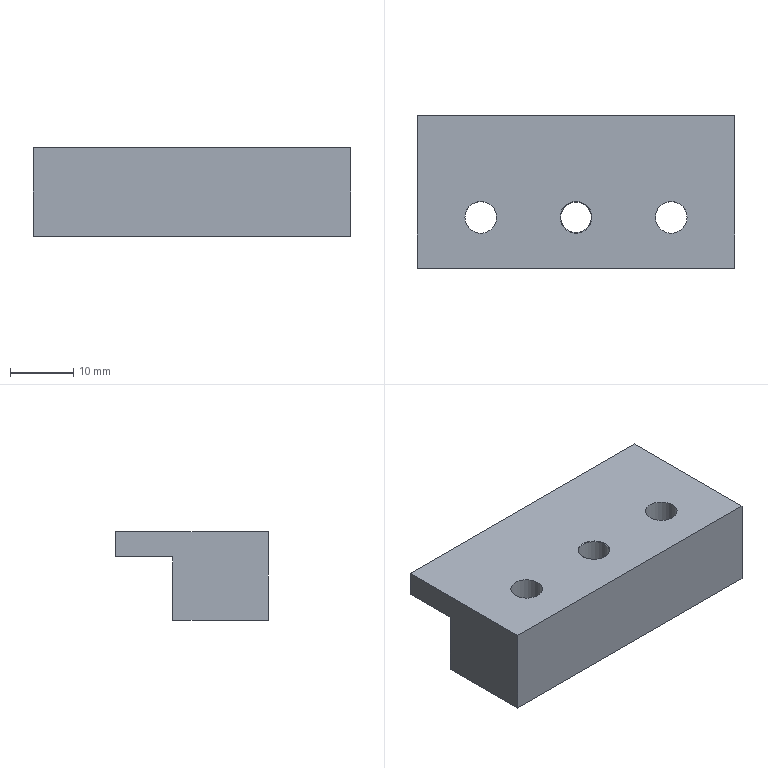Component | NX | GUIDE_PLATE_2 | 1 solid | 12 faces | box 50 x 24 x 14 mm | volume 11494 mm3 | plane 8 | cylinder 3 | cone 1 | commonest cylinder face diameters 5 x2 4.826 x1
STEP:
#1=CARTESIAN_POINT('',(0.,0.,0.));
#2=DIRECTION('',(0.,0.,1.));
#3=DIRECTION('',(1.,0.,0.));
#4=AXIS2_PLACEMENT_3D('',#1,#2,#3);
#5=CARTESIAN_POINT('',(28.,-11.,10.));
#6=VERTEX_POINT('',#5);
#7=CARTESIAN_POINT('',(28.,-11.,14.));
#8=VERTEX_POINT('',#7);
#9=CARTESIAN_POINT('',(28.,-11.,0.));
#10=DIRECTION('',(0.,0.,1.));
#11=VECTOR('',#10,1.);
#12=LINE('',#9,#11);
#13=CARTESIAN_POINT('',(28.,-11.,0.));
#14=DIRECTION('',(-0.,1.,0.));
#15=DIRECTION('',(-1.,-0.,0.));
#16=AXIS2_PLACEMENT_3D('',#13,#14,#15);
#17=PLANE('',#16);
#18=CARTESIAN_POINT('',(0.,0.));
#19=DIRECTION('',(0.,1.));
#20=VECTOR('',#19,1.);
#21=LINE('',#18,#20);
#22=(GEOMETRIC_REPRESENTATION_CONTEXT(2)PARAMETRIC_REPRESENTATION_CONTEXT()REPRESENTATION_CONTEXT('',''));
#23=DEFINITIONAL_REPRESENTATION('',(#21),#22);
#24=PCURVE('',#17,#23);
#25=CARTESIAN_POINT('',(28.,-35.,0.));
#26=DIRECTION('',(1.,0.,0.));
#27=DIRECTION('',(-0.,1.,0.));
#28=AXIS2_PLACEMENT_3D('',#25,#26,#27);
#29=PLANE('',#28);
#30=CARTESIAN_POINT('',(24.,0.));
#31=DIRECTION('',(0.,1.));
#32=VECTOR('',#31,1.);
#33=LINE('',#30,#32);
#34=(GEOMETRIC_REPRESENTATION_CONTEXT(2)PARAMETRIC_REPRESENTATION_CONTEXT()REPRESENTATION_CONTEXT('',''));
#35=DEFINITIONAL_REPRESENTATION('',(#33),#34);
#36=PCURVE('',#29,#35);
#37=SURFACE_CURVE('',#12,(#24,#36),.PCURVE_S1.);
#38=EDGE_CURVE('',#6,#8,#37,.T.);
#39=ORIENTED_EDGE('',*,*,#38,.F.);
#40=CARTESIAN_POINT('',(-22.,-11.,10.));
#41=VERTEX_POINT('',#40);
#42=CARTESIAN_POINT('',(55.,-11.,10.));
#43=DIRECTION('',(-1.,0.,0.));
#44=VECTOR('',#43,1.);
#45=LINE('',#42,#44);
#46=CARTESIAN_POINT('',(-27.,10.));
#47=DIRECTION('',(1.,0.));
#48=VECTOR('',#47,1.);
#49=LINE('',#46,#48);
#50=(GEOMETRIC_REPRESENTATION_CONTEXT(2)PARAMETRIC_REPRESENTATION_CONTEXT()REPRESENTATION_CONTEXT('',''));
#51=DEFINITIONAL_REPRESENTATION('',(#49),#50);
#52=PCURVE('',#17,#51);
#53=CARTESIAN_POINT('',(55.,-20.,10.));
#54=DIRECTION('',(0.,0.,1.));
#55=DIRECTION('',(0.,-1.,0.));
#56=AXIS2_PLACEMENT_3D('',#53,#54,#55);
#57=PLANE('',#56);
#58=CARTESIAN_POINT('',(-9.,0.));
#59=DIRECTION('',(0.,-1.));
#60=VECTOR('',#59,1.);
#61=LINE('',#58,#60);
#62=(GEOMETRIC_REPRESENTATION_CONTEXT(2)PARAMETRIC_REPRESENTATION_CONTEXT()REPRESENTATION_CONTEXT('',''));
#63=DEFINITIONAL_REPRESENTATION('',(#61),#62);
#64=PCURVE('',#57,#63);
#65=SURFACE_CURVE('',#45,(#52,#64),.PCURVE_S1.);
#66=EDGE_CURVE('',#6,#41,#65,.T.);
#67=ORIENTED_EDGE('',*,*,#66,.T.);
#68=CARTESIAN_POINT('',(-22.,-11.,14.));
#69=VERTEX_POINT('',#68);
#70=CARTESIAN_POINT('',(-22.,-11.,0.));
#71=DIRECTION('',(0.,0.,1.));
#72=VECTOR('',#71,1.);
#73=LINE('',#70,#72);
#74=CARTESIAN_POINT('',(50.,0.));
#75=DIRECTION('',(0.,1.));
#76=VECTOR('',#75,1.);
#77=LINE('',#74,#76);
#78=(GEOMETRIC_REPRESENTATION_CONTEXT(2)PARAMETRIC_REPRESENTATION_CONTEXT()REPRESENTATION_CONTEXT('',''));
#79=DEFINITIONAL_REPRESENTATION('',(#77),#78);
#80=PCURVE('',#17,#79);
#81=CARTESIAN_POINT('',(-22.,-11.,0.));
#82=DIRECTION('',(-1.,-0.,0.));
#83=DIRECTION('',(0.,-1.,0.));
#84=AXIS2_PLACEMENT_3D('',#81,#82,#83);
#85=PLANE('',#84);
#86=CARTESIAN_POINT('',(0.,0.));
#87=DIRECTION('',(0.,1.));
#88=VECTOR('',#87,1.);
#89=LINE('',#86,#88);
#90=(GEOMETRIC_REPRESENTATION_CONTEXT(2)PARAMETRIC_REPRESENTATION_CONTEXT()REPRESENTATION_CONTEXT('',''));
#91=DEFINITIONAL_REPRESENTATION('',(#89),#90);
#92=PCURVE('',#85,#91);
#93=SURFACE_CURVE('',#73,(#80,#92),.PCURVE_S1.);
#94=EDGE_CURVE('',#41,#69,#93,.T.);
#95=ORIENTED_EDGE('',*,*,#94,.T.);
#96=CARTESIAN_POINT('',(28.,-11.,14.));
#97=DIRECTION('',(-1.,-0.,0.));
#98=VECTOR('',#97,1.);
#99=LINE('',#96,#98);
#100=CARTESIAN_POINT('',(0.,14.));
#101=DIRECTION('',(1.,0.));
#102=VECTOR('',#101,1.);
#103=LINE('',#100,#102);
#104=(GEOMETRIC_REPRESENTATION_CONTEXT(2)PARAMETRIC_REPRESENTATION_CONTEXT()REPRESENTATION_CONTEXT('',''));
#105=DEFINITIONAL_REPRESENTATION('',(#103),#104);
#106=PCURVE('',#17,#105);
#107=CARTESIAN_POINT('',(-22.,-35.,14.));
#108=DIRECTION('',(0.,0.,1.));
#109=DIRECTION('',(1.,0.,0.));
#110=AXIS2_PLACEMENT_3D('',#107,#108,#109);
#111=PLANE('',#110);
#112=CARTESIAN_POINT('',(50.,24.));
#113=DIRECTION('',(-1.,-0.));
#114=VECTOR('',#113,1.);
#115=LINE('',#112,#114);
#116=(GEOMETRIC_REPRESENTATION_CONTEXT(2)PARAMETRIC_REPRESENTATION_CONTEXT()REPRESENTATION_CONTEXT('',''));
#117=DEFINITIONAL_REPRESENTATION('',(#115),#116);
#118=PCURVE('',#111,#117);
#119=SURFACE_CURVE('',#99,(#106,#118),.PCURVE_S1.);
#120=EDGE_CURVE('',#8,#69,#119,.T.);
#121=ORIENTED_EDGE('',*,*,#120,.F.);
#122=EDGE_LOOP('',(#39,#67,#95,#121));
#123=FACE_BOUND('',#122,.T.);
#124=ADVANCED_FACE('',(#123),#17,.T.);
#125=CARTESIAN_POINT('',(-9.5,-27.,0.));
#126=VERTEX_POINT('',#125);
#127=CARTESIAN_POINT('',(-14.5,-27.,0.));
#128=VERTEX_POINT('',#127);
#129=CARTESIAN_POINT('',(-12.,-27.,0.));
#130=DIRECTION('',(0.,0.,1.));
#131=DIRECTION('',(1.,0.,0.));
#132=AXIS2_PLACEMENT_3D('',#129,#130,#131);
#133=CIRCLE('',#132,2.5);
#134=CARTESIAN_POINT('',(-22.,-35.,0.));
#135=DIRECTION('',(0.,0.,1.));
#136=DIRECTION('',(1.,0.,0.));
#137=AXIS2_PLACEMENT_3D('',#134,#135,#136);
#138=PLANE('',#137);
#139=CARTESIAN_POINT('',(10.,8.));
#140=DIRECTION('',(1.,0.));
#141=AXIS2_PLACEMENT_2D('',#139,#140);
#142=CIRCLE('',#141,2.5);
#143=(GEOMETRIC_REPRESENTATION_CONTEXT(2)PARAMETRIC_REPRESENTATION_CONTEXT()REPRESENTATION_CONTEXT('',''));
#144=DEFINITIONAL_REPRESENTATION('',(#142),#143);
#145=PCURVE('',#138,#144);
#146=CARTESIAN_POINT('',(-12.,-27.,14.));
#147=DIRECTION('',(0.,0.,-1.));
#148=DIRECTION('',(-1.,0.,0.));
#149=AXIS2_PLACEMENT_3D('',#146,#147,#148);
#150=CYLINDRICAL_SURFACE('',#149,2.5);
#151=CARTESIAN_POINT('',(3.142,14.));
#152=DIRECTION('',(-1.,0.));
#153=VECTOR('',#152,1.);
#154=LINE('',#151,#153);
#155=(GEOMETRIC_REPRESENTATION_CONTEXT(2)PARAMETRIC_REPRESENTATION_CONTEXT()REPRESENTATION_CONTEXT('',''));
#156=DEFINITIONAL_REPRESENTATION('',(#154),#155);
#157=PCURVE('',#150,#156);
#158=SURFACE_CURVE('',#133,(#145,#157),.PCURVE_S1.);
#159=EDGE_CURVE('',#126,#128,#158,.T.);
#160=ORIENTED_EDGE('',*,*,#159,.T.);
#161=CARTESIAN_POINT('',(-12.,-27.,0.));
#162=DIRECTION('',(0.,0.,1.));
#163=DIRECTION('',(1.,0.,0.));
#164=AXIS2_PLACEMENT_3D('',#161,#162,#163);
#165=CIRCLE('',#164,2.5);
#166=CARTESIAN_POINT('',(10.,8.));
#167=DIRECTION('',(1.,0.));
#168=AXIS2_PLACEMENT_2D('',#166,#167);
#169=CIRCLE('',#168,2.5);
#170=(GEOMETRIC_REPRESENTATION_CONTEXT(2)PARAMETRIC_REPRESENTATION_CONTEXT()REPRESENTATION_CONTEXT('',''));
#171=DEFINITIONAL_REPRESENTATION('',(#169),#170);
#172=PCURVE('',#138,#171);
#173=CARTESIAN_POINT('',(9.425,14.));
#174=DIRECTION('',(-1.,0.));
#175=VECTOR('',#174,1.);
#176=LINE('',#173,#175);
#177=(GEOMETRIC_REPRESENTATION_CONTEXT(2)PARAMETRIC_REPRESENTATION_CONTEXT()REPRESENTATION_CONTEXT('',''));
#178=DEFINITIONAL_REPRESENTATION('',(#176),#177);
#179=PCURVE('',#150,#178);
#180=SURFACE_CURVE('',#165,(#172,#179),.PCURVE_S1.);
#181=EDGE_CURVE('',#128,#126,#180,.T.);
#182=ORIENTED_EDGE('',*,*,#181,.T.);
#183=EDGE_LOOP('',(#160,#182));
#184=FACE_BOUND('',#183,.T.);
#185=CARTESIAN_POINT('',(20.5,-27.,0.));
#186=VERTEX_POINT('',#185);
#187=CARTESIAN_POINT('',(15.5,-27.,0.));
#188=VERTEX_POINT('',#187);
#189=CARTESIAN_POINT('',(18.,-27.,0.));
#190=DIRECTION('',(0.,0.,1.));
#191=DIRECTION('',(1.,0.,0.));
#192=AXIS2_PLACEMENT_3D('',#189,#190,#191);
#193=CIRCLE('',#192,2.5);
#194=CARTESIAN_POINT('',(40.,8.));
#195=DIRECTION('',(1.,0.));
#196=AXIS2_PLACEMENT_2D('',#194,#195);
#197=CIRCLE('',#196,2.5);
#198=(GEOMETRIC_REPRESENTATION_CONTEXT(2)PARAMETRIC_REPRESENTATION_CONTEXT()REPRESENTATION_CONTEXT('',''));
#199=DEFINITIONAL_REPRESENTATION('',(#197),#198);
#200=PCURVE('',#138,#199);
#201=CARTESIAN_POINT('',(18.,-27.,14.));
#202=DIRECTION('',(0.,0.,-1.));
#203=DIRECTION('',(-1.,0.,0.));
#204=AXIS2_PLACEMENT_3D('',#201,#202,#203);
#205=CYLINDRICAL_SURFACE('',#204,2.5);
#206=CARTESIAN_POINT('',(3.142,14.));
#207=DIRECTION('',(-1.,0.));
#208=VECTOR('',#207,1.);
#209=LINE('',#206,#208);
#210=(GEOMETRIC_REPRESENTATION_CONTEXT(2)PARAMETRIC_REPRESENTATION_CONTEXT()REPRESENTATION_CONTEXT('',''));
#211=DEFINITIONAL_REPRESENTATION('',(#209),#210);
#212=PCURVE('',#205,#211);
#213=SURFACE_CURVE('',#193,(#200,#212),.PCURVE_S1.);
#214=EDGE_CURVE('',#186,#188,#213,.T.);
#215=ORIENTED_EDGE('',*,*,#214,.T.);
#216=CARTESIAN_POINT('',(18.,-27.,0.));
#217=DIRECTION('',(0.,0.,1.));
#218=DIRECTION('',(1.,0.,0.));
#219=AXIS2_PLACEMENT_3D('',#216,#217,#218);
#220=CIRCLE('',#219,2.5);
#221=CARTESIAN_POINT('',(40.,8.));
#222=DIRECTION('',(1.,0.));
#223=AXIS2_PLACEMENT_2D('',#221,#222);
#224=CIRCLE('',#223,2.5);
#225=(GEOMETRIC_REPRESENTATION_CONTEXT(2)PARAMETRIC_REPRESENTATION_CONTEXT()REPRESENTATION_CONTEXT('',''));
#226=DEFINITIONAL_REPRESENTATION('',(#224),#225);
#227=PCURVE('',#138,#226);
#228=CARTESIAN_POINT('',(9.425,14.));
#229=DIRECTION('',(-1.,0.));
#230=VECTOR('',#229,1.);
#231=LINE('',#228,#230);
#232=(GEOMETRIC_REPRESENTATION_CONTEXT(2)PARAMETRIC_REPRESENTATION_CONTEXT()REPRESENTATION_CONTEXT('',''));
#233=DEFINITIONAL_REPRESENTATION('',(#231),#232);
#234=PCURVE('',#205,#233);
#235=SURFACE_CURVE('',#220,(#227,#234),.PCURVE_S1.);
#236=EDGE_CURVE('',#188,#186,#235,.T.);
#237=ORIENTED_EDGE('',*,*,#236,.T.);
#238=EDGE_LOOP('',(#215,#237));
#239=FACE_BOUND('',#238,.T.);
#240=CARTESIAN_POINT('',(5.413,-27.,0.));
#241=VERTEX_POINT('',#240);
#242=CARTESIAN_POINT('',(3.,-27.,0.));
#243=DIRECTION('',(0.,0.,1.));
#244=DIRECTION('',(1.,0.,0.));
#245=AXIS2_PLACEMENT_3D('',#242,#243,#244);
#246=CIRCLE('',#245,2.413);
#247=CARTESIAN_POINT('',(25.,8.));
#248=DIRECTION('',(1.,0.));
#249=AXIS2_PLACEMENT_2D('',#247,#248);
#250=CIRCLE('',#249,2.413);
#251=(GEOMETRIC_REPRESENTATION_CONTEXT(2)PARAMETRIC_REPRESENTATION_CONTEXT()REPRESENTATION_CONTEXT('',''));
#252=DEFINITIONAL_REPRESENTATION('',(#250),#251);
#253=PCURVE('',#138,#252);
#254=CARTESIAN_POINT('',(3.,-27.,14.));
#255=DIRECTION('',(0.,0.,-1.));
#256=DIRECTION('',(-1.,0.,0.));
#257=AXIS2_PLACEMENT_3D('',#254,#255,#256);
#258=CYLINDRICAL_SURFACE('',#257,2.413);
#259=CARTESIAN_POINT('',(9.425,14.));
#260=DIRECTION('',(-1.,0.));
#261=VECTOR('',#260,1.);
#262=LINE('',#259,#261);
#263=(GEOMETRIC_REPRESENTATION_CONTEXT(2)PARAMETRIC_REPRESENTATION_CONTEXT()REPRESENTATION_CONTEXT('',''));
#264=DEFINITIONAL_REPRESENTATION('',(#262),#263);
#265=PCURVE('',#258,#264);
#266=SURFACE_CURVE('',#246,(#253,#265),.PCURVE_S1.);
#267=EDGE_CURVE('',#241,#241,#266,.T.);
#268=ORIENTED_EDGE('',*,*,#267,.T.);
#269=EDGE_LOOP('',(#268));
#270=FACE_BOUND('',#269,.T.);
#271=CARTESIAN_POINT('',(28.,-20.,0.));
#272=VERTEX_POINT('',#271);
#273=CARTESIAN_POINT('',(-22.,-20.,0.));
#274=VERTEX_POINT('',#273);
#275=CARTESIAN_POINT('',(55.,-20.,0.));
#276=DIRECTION('',(-1.,0.,0.));
#277=VECTOR('',#276,1.);
#278=LINE('',#275,#277);
#279=CARTESIAN_POINT('',(77.,15.));
#280=DIRECTION('',(-1.,0.));
#281=VECTOR('',#280,1.);
#282=LINE('',#279,#281);
#283=(GEOMETRIC_REPRESENTATION_CONTEXT(2)PARAMETRIC_REPRESENTATION_CONTEXT()REPRESENTATION_CONTEXT('',''));
#284=DEFINITIONAL_REPRESENTATION('',(#282),#283);
#285=PCURVE('',#138,#284);
#286=CARTESIAN_POINT('',(55.,-20.,0.));
#287=DIRECTION('',(0.,-1.,0.));
#288=DIRECTION('',(0.,-0.,-1.));
#289=AXIS2_PLACEMENT_3D('',#286,#287,#288);
#290=PLANE('',#289);
#291=CARTESIAN_POINT('',(0.,0.));
#292=DIRECTION('',(0.,-1.));
#293=VECTOR('',#292,1.);
#294=LINE('',#291,#293);
#295=(GEOMETRIC_REPRESENTATION_CONTEXT(2)PARAMETRIC_REPRESENTATION_CONTEXT()REPRESENTATION_CONTEXT('',''));
#296=DEFINITIONAL_REPRESENTATION('',(#294),#295);
#297=PCURVE('',#290,#296);
#298=SURFACE_CURVE('',#278,(#285,#297),.PCURVE_S1.);
#299=EDGE_CURVE('',#272,#274,#298,.T.);
#300=ORIENTED_EDGE('',*,*,#299,.F.);
#301=CARTESIAN_POINT('',(28.,-35.,0.));
#302=VERTEX_POINT('',#301);
#303=CARTESIAN_POINT('',(28.,-35.,0.));
#304=DIRECTION('',(-0.,1.,0.));
#305=VECTOR('',#304,1.);
#306=LINE('',#303,#305);
#307=CARTESIAN_POINT('',(50.,0.));
#308=DIRECTION('',(-0.,1.));
#309=VECTOR('',#308,1.);
#310=LINE('',#307,#309);
#311=(GEOMETRIC_REPRESENTATION_CONTEXT(2)PARAMETRIC_REPRESENTATION_CONTEXT()REPRESENTATION_CONTEXT('',''));
#312=DEFINITIONAL_REPRESENTATION('',(#310),#311);
#313=PCURVE('',#138,#312);
#314=CARTESIAN_POINT('',(0.,0.));
#315=DIRECTION('',(1.,0.));
#316=VECTOR('',#315,1.);
#317=LINE('',#314,#316);
#318=(GEOMETRIC_REPRESENTATION_CONTEXT(2)PARAMETRIC_REPRESENTATION_CONTEXT()REPRESENTATION_CONTEXT('',''));
#319=DEFINITIONAL_REPRESENTATION('',(#317),#318);
#320=PCURVE('',#29,#319);
#321=SURFACE_CURVE('',#306,(#313,#320),.PCURVE_S1.);
#322=EDGE_CURVE('',#302,#272,#321,.T.);
#323=ORIENTED_EDGE('',*,*,#322,.F.);
#324=CARTESIAN_POINT('',(-22.,-35.,0.));
#325=VERTEX_POINT('',#324);
#326=CARTESIAN_POINT('',(-22.,-35.,0.));
#327=DIRECTION('',(1.,-0.,0.));
#328=VECTOR('',#327,1.);
#329=LINE('',#326,#328);
#330=CARTESIAN_POINT('',(0.,0.));
#331=DIRECTION('',(1.,-0.));
#332=VECTOR('',#331,1.);
#333=LINE('',#330,#332);
#334=(GEOMETRIC_REPRESENTATION_CONTEXT(2)PARAMETRIC_REPRESENTATION_CONTEXT()REPRESENTATION_CONTEXT('',''));
#335=DEFINITIONAL_REPRESENTATION('',(#333),#334);
#336=PCURVE('',#138,#335);
#337=CARTESIAN_POINT('',(-22.,-35.,0.));
#338=DIRECTION('',(-0.,-1.,0.));
#339=DIRECTION('',(1.,-0.,0.));
#340=AXIS2_PLACEMENT_3D('',#337,#338,#339);
#341=PLANE('',#340);
#342=CARTESIAN_POINT('',(0.,0.));
#343=DIRECTION('',(1.,0.));
#344=VECTOR('',#343,1.);
#345=LINE('',#342,#344);
#346=(GEOMETRIC_REPRESENTATION_CONTEXT(2)PARAMETRIC_REPRESENTATION_CONTEXT()REPRESENTATION_CONTEXT('',''));
#347=DEFINITIONAL_REPRESENTATION('',(#345),#346);
#348=PCURVE('',#341,#347);
#349=SURFACE_CURVE('',#329,(#336,#348),.PCURVE_S1.);
#350=EDGE_CURVE('',#325,#302,#349,.T.);
#351=ORIENTED_EDGE('',*,*,#350,.F.);
#352=CARTESIAN_POINT('',(-22.,-11.,0.));
#353=DIRECTION('',(0.,-1.,0.));
#354=VECTOR('',#353,1.);
#355=LINE('',#352,#354);
#356=CARTESIAN_POINT('',(0.,24.));
#357=DIRECTION('',(0.,-1.));
#358=VECTOR('',#357,1.);
#359=LINE('',#356,#358);
#360=(GEOMETRIC_REPRESENTATION_CONTEXT(2)PARAMETRIC_REPRESENTATION_CONTEXT()REPRESENTATION_CONTEXT('',''));
#361=DEFINITIONAL_REPRESENTATION('',(#359),#360);
#362=PCURVE('',#138,#361);
#363=CARTESIAN_POINT('',(0.,0.));
#364=DIRECTION('',(1.,0.));
#365=VECTOR('',#364,1.);
#366=LINE('',#363,#365);
#367=(GEOMETRIC_REPRESENTATION_CONTEXT(2)PARAMETRIC_REPRESENTATION_CONTEXT()REPRESENTATION_CONTEXT('',''));
#368=DEFINITIONAL_REPRESENTATION('',(#366),#367);
#369=PCURVE('',#85,#368);
#370=SURFACE_CURVE('',#355,(#362,#369),.PCURVE_S1.);
#371=EDGE_CURVE('',#274,#325,#370,.T.);
#372=ORIENTED_EDGE('',*,*,#371,.F.);
#373=EDGE_LOOP('',(#300,#323,#351,#372));
#374=FACE_BOUND('',#373,.T.);
#375=ADVANCED_FACE('',(#184,#239,#270,#374),#138,.F.);
#376=CARTESIAN_POINT('',(-22.,-20.,10.));
#377=VERTEX_POINT('',#376);
#378=CARTESIAN_POINT('',(-22.,-20.,0.));
#379=DIRECTION('',(-0.,0.,1.));
#380=VECTOR('',#379,1.);
#381=LINE('',#378,#380);
#382=CARTESIAN_POINT('',(9.,0.));
#383=DIRECTION('',(-0.,1.));
#384=VECTOR('',#383,1.);
#385=LINE('',#382,#384);
#386=(GEOMETRIC_REPRESENTATION_CONTEXT(2)PARAMETRIC_REPRESENTATION_CONTEXT()REPRESENTATION_CONTEXT('',''));
#387=DEFINITIONAL_REPRESENTATION('',(#385),#386);
#388=PCURVE('',#85,#387);
#389=CARTESIAN_POINT('',(-0.,-77.));
#390=DIRECTION('',(-1.,-0.));
#391=VECTOR('',#390,1.);
#392=LINE('',#389,#391);
#393=(GEOMETRIC_REPRESENTATION_CONTEXT(2)PARAMETRIC_REPRESENTATION_CONTEXT()REPRESENTATION_CONTEXT('',''));
#394=DEFINITIONAL_REPRESENTATION('',(#392),#393);
#395=PCURVE('',#290,#394);
#396=SURFACE_CURVE('',#381,(#388,#395),.PCURVE_S1.);
#397=EDGE_CURVE('',#274,#377,#396,.T.);
#398=ORIENTED_EDGE('',*,*,#397,.F.);
#399=ORIENTED_EDGE('',*,*,#371,.T.);
#400=CARTESIAN_POINT('',(-22.,-35.,14.));
#401=VERTEX_POINT('',#400);
#402=CARTESIAN_POINT('',(-22.,-35.,0.));
#403=DIRECTION('',(0.,0.,1.));
#404=VECTOR('',#403,1.);
#405=LINE('',#402,#404);
#406=CARTESIAN_POINT('',(24.,0.));
#407=DIRECTION('',(0.,1.));
#408=VECTOR('',#407,1.);
#409=LINE('',#406,#408);
#410=(GEOMETRIC_REPRESENTATION_CONTEXT(2)PARAMETRIC_REPRESENTATION_CONTEXT()REPRESENTATION_CONTEXT('',''));
#411=DEFINITIONAL_REPRESENTATION('',(#409),#410);
#412=PCURVE('',#85,#411);
#413=CARTESIAN_POINT('',(0.,0.));
#414=DIRECTION('',(0.,1.));
#415=VECTOR('',#414,1.);
#416=LINE('',#413,#415);
#417=(GEOMETRIC_REPRESENTATION_CONTEXT(2)PARAMETRIC_REPRESENTATION_CONTEXT()REPRESENTATION_CONTEXT('',''));
#418=DEFINITIONAL_REPRESENTATION('',(#416),#417);
#419=PCURVE('',#341,#418);
#420=SURFACE_CURVE('',#405,(#412,#419),.PCURVE_S1.);
#421=EDGE_CURVE('',#325,#401,#420,.T.);
#422=ORIENTED_EDGE('',*,*,#421,.T.);
#423=CARTESIAN_POINT('',(-22.,-11.,14.));
#424=DIRECTION('',(0.,-1.,0.));
#425=VECTOR('',#424,1.);
#426=LINE('',#423,#425);
#427=CARTESIAN_POINT('',(0.,14.));
#428=DIRECTION('',(1.,0.));
#429=VECTOR('',#428,1.);
#430=LINE('',#427,#429);
#431=(GEOMETRIC_REPRESENTATION_CONTEXT(2)PARAMETRIC_REPRESENTATION_CONTEXT()REPRESENTATION_CONTEXT('',''));
#432=DEFINITIONAL_REPRESENTATION('',(#430),#431);
#433=PCURVE('',#85,#432);
#434=CARTESIAN_POINT('',(0.,24.));
#435=DIRECTION('',(0.,-1.));
#436=VECTOR('',#435,1.);
#437=LINE('',#434,#436);
#438=(GEOMETRIC_REPRESENTATION_CONTEXT(2)PARAMETRIC_REPRESENTATION_CONTEXT()REPRESENTATION_CONTEXT('',''));
#439=DEFINITIONAL_REPRESENTATION('',(#437),#438);
#440=PCURVE('',#111,#439);
#441=SURFACE_CURVE('',#426,(#433,#440),.PCURVE_S1.);
#442=EDGE_CURVE('',#69,#401,#441,.T.);
#443=ORIENTED_EDGE('',*,*,#442,.F.);
#444=ORIENTED_EDGE('',*,*,#94,.F.);
#445=CARTESIAN_POINT('',(-22.,-11.,10.));
#446=DIRECTION('',(-0.,1.,-0.));
#447=VECTOR('',#446,1.);
#448=LINE('',#445,#447);
#449=CARTESIAN_POINT('',(0.,10.));
#450=DIRECTION('',(-1.,-0.));
#451=VECTOR('',#450,1.);
#452=LINE('',#449,#451);
#453=(GEOMETRIC_REPRESENTATION_CONTEXT(2)PARAMETRIC_REPRESENTATION_CONTEXT()REPRESENTATION_CONTEXT('',''));
#454=DEFINITIONAL_REPRESENTATION('',(#452),#453);
#455=PCURVE('',#85,#454);
#456=CARTESIAN_POINT('',(-9.,-77.));
#457=DIRECTION('',(-1.,-0.));
#458=VECTOR('',#457,1.);
#459=LINE('',#456,#458);
#460=(GEOMETRIC_REPRESENTATION_CONTEXT(2)PARAMETRIC_REPRESENTATION_CONTEXT()REPRESENTATION_CONTEXT('',''));
#461=DEFINITIONAL_REPRESENTATION('',(#459),#460);
#462=PCURVE('',#57,#461);
#463=SURFACE_CURVE('',#448,(#455,#462),.PCURVE_S1.);
#464=EDGE_CURVE('',#377,#41,#463,.T.);
#465=ORIENTED_EDGE('',*,*,#464,.F.);
#466=EDGE_LOOP('',(#398,#399,#422,#443,#444,#465));
#467=FACE_BOUND('',#466,.T.);
#468=ADVANCED_FACE('',(#467),#85,.T.);
#469=CARTESIAN_POINT('',(28.,-35.,14.));
#470=VERTEX_POINT('',#469);
#471=CARTESIAN_POINT('',(-22.,-35.,14.));
#472=DIRECTION('',(1.,-0.,0.));
#473=VECTOR('',#472,1.);
#474=LINE('',#471,#473);
#475=CARTESIAN_POINT('',(0.,14.));
#476=DIRECTION('',(1.,0.));
#477=VECTOR('',#476,1.);
#478=LINE('',#475,#477);
#479=(GEOMETRIC_REPRESENTATION_CONTEXT(2)PARAMETRIC_REPRESENTATION_CONTEXT()REPRESENTATION_CONTEXT('',''));
#480=DEFINITIONAL_REPRESENTATION('',(#478),#479);
#481=PCURVE('',#341,#480);
#482=CARTESIAN_POINT('',(0.,0.));
#483=DIRECTION('',(1.,-0.));
#484=VECTOR('',#483,1.);
#485=LINE('',#482,#484);
#486=(GEOMETRIC_REPRESENTATION_CONTEXT(2)PARAMETRIC_REPRESENTATION_CONTEXT()REPRESENTATION_CONTEXT('',''));
#487=DEFINITIONAL_REPRESENTATION('',(#485),#486);
#488=PCURVE('',#111,#487);
#489=SURFACE_CURVE('',#474,(#481,#488),.PCURVE_S1.);
#490=EDGE_CURVE('',#401,#470,#489,.T.);
#491=ORIENTED_EDGE('',*,*,#490,.F.);
#492=ORIENTED_EDGE('',*,*,#421,.F.);
#493=ORIENTED_EDGE('',*,*,#350,.T.);
#494=CARTESIAN_POINT('',(28.,-35.,0.));
#495=DIRECTION('',(0.,0.,1.));
#496=VECTOR('',#495,1.);
#497=LINE('',#494,#496);
#498=CARTESIAN_POINT('',(50.,0.));
#499=DIRECTION('',(0.,1.));
#500=VECTOR('',#499,1.);
#501=LINE('',#498,#500);
#502=(GEOMETRIC_REPRESENTATION_CONTEXT(2)PARAMETRIC_REPRESENTATION_CONTEXT()REPRESENTATION_CONTEXT('',''));
#503=DEFINITIONAL_REPRESENTATION('',(#501),#502);
#504=PCURVE('',#341,#503);
#505=CARTESIAN_POINT('',(0.,0.));
#506=DIRECTION('',(0.,1.));
#507=VECTOR('',#506,1.);
#508=LINE('',#505,#507);
#509=(GEOMETRIC_REPRESENTATION_CONTEXT(2)PARAMETRIC_REPRESENTATION_CONTEXT()REPRESENTATION_CONTEXT('',''));
#510=DEFINITIONAL_REPRESENTATION('',(#508),#509);
#511=PCURVE('',#29,#510);
#512=SURFACE_CURVE('',#497,(#504,#511),.PCURVE_S1.);
#513=EDGE_CURVE('',#302,#470,#512,.T.);
#514=ORIENTED_EDGE('',*,*,#513,.T.);
#515=EDGE_LOOP('',(#491,#492,#493,#514));
#516=FACE_BOUND('',#515,.T.);
#517=ADVANCED_FACE('',(#516),#341,.T.);
#518=CARTESIAN_POINT('',(28.,-20.,10.));
#519=VERTEX_POINT('',#518);
#520=CARTESIAN_POINT('',(28.,-20.,-0.));
#521=DIRECTION('',(0.,-0.,-1.));
#522=VECTOR('',#521,1.);
#523=LINE('',#520,#522);
#524=CARTESIAN_POINT('',(15.,-0.));
#525=DIRECTION('',(-0.,-1.));
#526=VECTOR('',#525,1.);
#527=LINE('',#524,#526);
#528=(GEOMETRIC_REPRESENTATION_CONTEXT(2)PARAMETRIC_REPRESENTATION_CONTEXT()REPRESENTATION_CONTEXT('',''));
#529=DEFINITIONAL_REPRESENTATION('',(#527),#528);
#530=PCURVE('',#29,#529);
#531=CARTESIAN_POINT('',(0.,-27.));
#532=DIRECTION('',(1.,0.));
#533=VECTOR('',#532,1.);
#534=LINE('',#531,#533);
#535=(GEOMETRIC_REPRESENTATION_CONTEXT(2)PARAMETRIC_REPRESENTATION_CONTEXT()REPRESENTATION_CONTEXT('',''));
#536=DEFINITIONAL_REPRESENTATION('',(#534),#535);
#537=PCURVE('',#290,#536);
#538=SURFACE_CURVE('',#523,(#530,#537),.PCURVE_S1.);
#539=EDGE_CURVE('',#519,#272,#538,.T.);
#540=ORIENTED_EDGE('',*,*,#539,.F.);
#541=CARTESIAN_POINT('',(28.,-35.,10.));
#542=DIRECTION('',(0.,-1.,0.));
#543=VECTOR('',#542,1.);
#544=LINE('',#541,#543);
#545=CARTESIAN_POINT('',(0.,10.));
#546=DIRECTION('',(-1.,0.));
#547=VECTOR('',#546,1.);
#548=LINE('',#545,#547);
#549=(GEOMETRIC_REPRESENTATION_CONTEXT(2)PARAMETRIC_REPRESENTATION_CONTEXT()REPRESENTATION_CONTEXT('',''));
#550=DEFINITIONAL_REPRESENTATION('',(#548),#549);
#551=PCURVE('',#29,#550);
#552=CARTESIAN_POINT('',(15.,-27.));
#553=DIRECTION('',(1.,0.));
#554=VECTOR('',#553,1.);
#555=LINE('',#552,#554);
#556=(GEOMETRIC_REPRESENTATION_CONTEXT(2)PARAMETRIC_REPRESENTATION_CONTEXT()REPRESENTATION_CONTEXT('',''));
#557=DEFINITIONAL_REPRESENTATION('',(#555),#556);
#558=PCURVE('',#57,#557);
#559=SURFACE_CURVE('',#544,(#551,#558),.PCURVE_S1.);
#560=EDGE_CURVE('',#6,#519,#559,.T.);
#561=ORIENTED_EDGE('',*,*,#560,.F.);
#562=ORIENTED_EDGE('',*,*,#38,.T.);
#563=CARTESIAN_POINT('',(28.,-35.,14.));
#564=DIRECTION('',(-0.,1.,0.));
#565=VECTOR('',#564,1.);
#566=LINE('',#563,#565);
#567=CARTESIAN_POINT('',(0.,14.));
#568=DIRECTION('',(1.,0.));
#569=VECTOR('',#568,1.);
#570=LINE('',#567,#569);
#571=(GEOMETRIC_REPRESENTATION_CONTEXT(2)PARAMETRIC_REPRESENTATION_CONTEXT()REPRESENTATION_CONTEXT('',''));
#572=DEFINITIONAL_REPRESENTATION('',(#570),#571);
#573=PCURVE('',#29,#572);
#574=CARTESIAN_POINT('',(50.,0.));
#575=DIRECTION('',(-0.,1.));
#576=VECTOR('',#575,1.);
#577=LINE('',#574,#576);
#578=(GEOMETRIC_REPRESENTATION_CONTEXT(2)PARAMETRIC_REPRESENTATION_CONTEXT()REPRESENTATION_CONTEXT('',''));
#579=DEFINITIONAL_REPRESENTATION('',(#577),#578);
#580=PCURVE('',#111,#579);
#581=SURFACE_CURVE('',#566,(#573,#580),.PCURVE_S1.);
#582=EDGE_CURVE('',#470,#8,#581,.T.);
#583=ORIENTED_EDGE('',*,*,#582,.F.);
#584=ORIENTED_EDGE('',*,*,#513,.F.);
#585=ORIENTED_EDGE('',*,*,#322,.T.);
#586=EDGE_LOOP('',(#540,#561,#562,#583,#584,#585));
#587=FACE_BOUND('',#586,.T.);
#588=ADVANCED_FACE('',(#587),#29,.T.);
#589=CARTESIAN_POINT('',(5.5,-27.,14.));
#590=VERTEX_POINT('',#589);
#591=CARTESIAN_POINT('',(3.,-27.,14.));
#592=DIRECTION('',(0.,0.,-1.));
#593=DIRECTION('',(1.,0.,0.));
#594=AXIS2_PLACEMENT_3D('',#591,#592,#593);
#595=CIRCLE('',#594,2.5);
#596=CARTESIAN_POINT('',(27.5,8.));
#597=CARTESIAN_POINT('',(27.5,3.67));
#598=CARTESIAN_POINT('',(23.75,5.835));
#599=CARTESIAN_POINT('',(20.,8.));
#600=CARTESIAN_POINT('',(23.75,10.165));
#601=CARTESIAN_POINT('',(27.5,12.33));
#602=CARTESIAN_POINT('',(27.5,8.));
#603=(BOUNDED_CURVE()B_SPLINE_CURVE(2,(#596,#597,#598,#599,#600,#601,#602),.UNSPECIFIED.,.T.,.F.)B_SPLINE_CURVE_WITH_KNOTS((1,2,2,2,2,1),(-2.094,0.,2.094,4.189,6.283,8.378),.UNSPECIFIED.)CURVE()GEOMETRIC_REPRESENTATION_ITEM()RATIONAL_B_SPLINE_CURVE((1.,0.5,1.,0.5,1.,0.5,1.))REPRESENTATION_ITEM(''));
#604=(GEOMETRIC_REPRESENTATION_CONTEXT(2)PARAMETRIC_REPRESENTATION_CONTEXT()REPRESENTATION_CONTEXT('',''));
#605=DEFINITIONAL_REPRESENTATION('',(#603),#604);
#606=PCURVE('',#111,#605);
#607=CARTESIAN_POINT('',(3.,-27.,14.));
#608=DIRECTION('',(0.,0.,1.));
#609=DIRECTION('',(1.,0.,0.));
#610=AXIS2_PLACEMENT_3D('',#607,#608,#609);
#611=CONICAL_SURFACE('',#610,2.5,0.7854);
#612=CARTESIAN_POINT('',(6.283,0.));
#613=DIRECTION('',(-1.,0.));
#614=VECTOR('',#613,1.);
#615=LINE('',#612,#614);
#616=(GEOMETRIC_REPRESENTATION_CONTEXT(2)PARAMETRIC_REPRESENTATION_CONTEXT()REPRESENTATION_CONTEXT('',''));
#617=DEFINITIONAL_REPRESENTATION('',(#615),#616);
#618=PCURVE('',#611,#617);
#619=SURFACE_CURVE('',#595,(#606,#618),.PCURVE_S1.);
#620=EDGE_CURVE('',#590,#590,#619,.T.);
#621=ORIENTED_EDGE('',*,*,#620,.T.);
#622=EDGE_LOOP('',(#621));
#623=FACE_BOUND('',#622,.T.);
#624=CARTESIAN_POINT('',(15.5,-27.,14.));
#625=VERTEX_POINT('',#624);
#626=CARTESIAN_POINT('',(18.,-27.,14.));
#627=DIRECTION('',(0.,0.,-1.));
#628=DIRECTION('',(-1.,0.,0.));
#629=AXIS2_PLACEMENT_3D('',#626,#627,#628);
#630=CIRCLE('',#629,2.5);
#631=CARTESIAN_POINT('',(37.5,8.));
#632=CARTESIAN_POINT('',(37.5,12.33));
#633=CARTESIAN_POINT('',(41.25,10.165));
#634=CARTESIAN_POINT('',(45.,8.));
#635=CARTESIAN_POINT('',(41.25,5.835));
#636=CARTESIAN_POINT('',(37.5,3.67));
#637=CARTESIAN_POINT('',(37.5,8.));
#638=(BOUNDED_CURVE()B_SPLINE_CURVE(2,(#631,#632,#633,#634,#635,#636,#637),.UNSPECIFIED.,.T.,.F.)B_SPLINE_CURVE_WITH_KNOTS((1,2,2,2,2,1),(-2.094,0.,2.094,4.189,6.283,8.378),.UNSPECIFIED.)CURVE()GEOMETRIC_REPRESENTATION_ITEM()RATIONAL_B_SPLINE_CURVE((1.,0.5,1.,0.5,1.,0.5,1.))REPRESENTATION_ITEM(''));
#639=(GEOMETRIC_REPRESENTATION_CONTEXT(2)PARAMETRIC_REPRESENTATION_CONTEXT()REPRESENTATION_CONTEXT('',''));
#640=DEFINITIONAL_REPRESENTATION('',(#638),#639);
#641=PCURVE('',#111,#640);
#642=CARTESIAN_POINT('',(0.,0.));
#643=DIRECTION('',(1.,0.));
#644=VECTOR('',#643,1.);
#645=LINE('',#642,#644);
#646=(GEOMETRIC_REPRESENTATION_CONTEXT(2)PARAMETRIC_REPRESENTATION_CONTEXT()REPRESENTATION_CONTEXT('',''));
#647=DEFINITIONAL_REPRESENTATION('',(#645),#646);
#648=PCURVE('',#205,#647);
#649=SURFACE_CURVE('',#630,(#641,#648),.PCURVE_S1.);
#650=EDGE_CURVE('',#625,#625,#649,.T.);
#651=ORIENTED_EDGE('',*,*,#650,.T.);
#652=EDGE_LOOP('',(#651));
#653=FACE_BOUND('',#652,.T.);
#654=CARTESIAN_POINT('',(-14.5,-27.,14.));
#655=VERTEX_POINT('',#654);
#656=CARTESIAN_POINT('',(-12.,-27.,14.));
#657=DIRECTION('',(0.,0.,-1.));
#658=DIRECTION('',(-1.,0.,0.));
#659=AXIS2_PLACEMENT_3D('',#656,#657,#658);
#660=CIRCLE('',#659,2.5);
#661=CARTESIAN_POINT('',(7.5,8.));
#662=CARTESIAN_POINT('',(7.5,12.33));
#663=CARTESIAN_POINT('',(11.25,10.165));
#664=CARTESIAN_POINT('',(15.,8.));
#665=CARTESIAN_POINT('',(11.25,5.835));
#666=CARTESIAN_POINT('',(7.5,3.67));
#667=CARTESIAN_POINT('',(7.5,8.));
#668=(BOUNDED_CURVE()B_SPLINE_CURVE(2,(#661,#662,#663,#664,#665,#666,#667),.UNSPECIFIED.,.T.,.F.)B_SPLINE_CURVE_WITH_KNOTS((1,2,2,2,2,1),(-2.094,0.,2.094,4.189,6.283,8.378),.UNSPECIFIED.)CURVE()GEOMETRIC_REPRESENTATION_ITEM()RATIONAL_B_SPLINE_CURVE((1.,0.5,1.,0.5,1.,0.5,1.))REPRESENTATION_ITEM(''));
#669=(GEOMETRIC_REPRESENTATION_CONTEXT(2)PARAMETRIC_REPRESENTATION_CONTEXT()REPRESENTATION_CONTEXT('',''));
#670=DEFINITIONAL_REPRESENTATION('',(#668),#669);
#671=PCURVE('',#111,#670);
#672=CARTESIAN_POINT('',(0.,0.));
#673=DIRECTION('',(1.,0.));
#674=VECTOR('',#673,1.);
#675=LINE('',#672,#674);
#676=(GEOMETRIC_REPRESENTATION_CONTEXT(2)PARAMETRIC_REPRESENTATION_CONTEXT()REPRESENTATION_CONTEXT('',''));
#677=DEFINITIONAL_REPRESENTATION('',(#675),#676);
#678=PCURVE('',#150,#677);
#679=SURFACE_CURVE('',#660,(#671,#678),.PCURVE_S1.);
#680=EDGE_CURVE('',#655,#655,#679,.T.);
#681=ORIENTED_EDGE('',*,*,#680,.T.);
#682=EDGE_LOOP('',(#681));
#683=FACE_BOUND('',#682,.T.);
#684=ORIENTED_EDGE('',*,*,#442,.T.);
#685=ORIENTED_EDGE('',*,*,#490,.T.);
#686=ORIENTED_EDGE('',*,*,#582,.T.);
#687=ORIENTED_EDGE('',*,*,#120,.T.);
#688=EDGE_LOOP('',(#684,#685,#686,#687));
#689=FACE_BOUND('',#688,.T.);
#690=ADVANCED_FACE('',(#623,#653,#683,#689),#111,.T.);
#691=ORIENTED_EDGE('',*,*,#680,.T.);
#692=CARTESIAN_POINT('',(-14.5,-27.,14.));
#693=CARTESIAN_POINT('',(-14.5,-27.,0.));
#694=B_SPLINE_CURVE_WITH_KNOTS('',1,(#692,#693),.UNSPECIFIED.,.F.,.F.,(2,2),(0.,14.),.PIECEWISE_BEZIER_KNOTS.);
#695=CARTESIAN_POINT('',(6.283,0.));
#696=DIRECTION('',(0.,1.));
#697=VECTOR('',#696,1.);
#698=LINE('',#695,#697);
#699=(GEOMETRIC_REPRESENTATION_CONTEXT(2)PARAMETRIC_REPRESENTATION_CONTEXT()REPRESENTATION_CONTEXT('',''));
#700=DEFINITIONAL_REPRESENTATION('',(#698),#699);
#701=PCURVE('',#150,#700);
#702=CARTESIAN_POINT('',(0.,0.));
#703=DIRECTION('',(0.,1.));
#704=VECTOR('',#703,1.);
#705=LINE('',#702,#704);
#706=(GEOMETRIC_REPRESENTATION_CONTEXT(2)PARAMETRIC_REPRESENTATION_CONTEXT()REPRESENTATION_CONTEXT('',''));
#707=DEFINITIONAL_REPRESENTATION('',(#705),#706);
#708=PCURVE('',#150,#707);
#709=SEAM_CURVE('',#694,(#701,#708),.PCURVE_S1.);
#710=EDGE_CURVE('',#655,#128,#709,.T.);
#711=ORIENTED_EDGE('',*,*,#710,.T.);
#712=ORIENTED_EDGE('',*,*,#181,.T.);
#713=ORIENTED_EDGE('',*,*,#159,.T.);
#714=ORIENTED_EDGE('',*,*,#710,.F.);
#715=EDGE_LOOP('',(#691,#711,#712,#713,#714));
#716=FACE_BOUND('',#715,.F.);
#717=ADVANCED_FACE('',(#716),#150,.F.);
#718=ORIENTED_EDGE('',*,*,#650,.T.);
#719=CARTESIAN_POINT('',(15.5,-27.,14.));
#720=CARTESIAN_POINT('',(15.5,-27.,0.));
#721=B_SPLINE_CURVE_WITH_KNOTS('',1,(#719,#720),.UNSPECIFIED.,.F.,.F.,(2,2),(0.,14.),.PIECEWISE_BEZIER_KNOTS.);
#722=CARTESIAN_POINT('',(6.283,0.));
#723=DIRECTION('',(0.,1.));
#724=VECTOR('',#723,1.);
#725=LINE('',#722,#724);
#726=(GEOMETRIC_REPRESENTATION_CONTEXT(2)PARAMETRIC_REPRESENTATION_CONTEXT()REPRESENTATION_CONTEXT('',''));
#727=DEFINITIONAL_REPRESENTATION('',(#725),#726);
#728=PCURVE('',#205,#727);
#729=CARTESIAN_POINT('',(0.,0.));
#730=DIRECTION('',(0.,1.));
#731=VECTOR('',#730,1.);
#732=LINE('',#729,#731);
#733=(GEOMETRIC_REPRESENTATION_CONTEXT(2)PARAMETRIC_REPRESENTATION_CONTEXT()REPRESENTATION_CONTEXT('',''));
#734=DEFINITIONAL_REPRESENTATION('',(#732),#733);
#735=PCURVE('',#205,#734);
#736=SEAM_CURVE('',#721,(#728,#735),.PCURVE_S1.);
#737=EDGE_CURVE('',#625,#188,#736,.T.);
#738=ORIENTED_EDGE('',*,*,#737,.T.);
#739=ORIENTED_EDGE('',*,*,#236,.T.);
#740=ORIENTED_EDGE('',*,*,#214,.T.);
#741=ORIENTED_EDGE('',*,*,#737,.F.);
#742=EDGE_LOOP('',(#718,#738,#739,#740,#741));
#743=FACE_BOUND('',#742,.F.);
#744=ADVANCED_FACE('',(#743),#205,.F.);
#745=CARTESIAN_POINT('',(5.413,-27.,13.913));
#746=VERTEX_POINT('',#745);
#747=CARTESIAN_POINT('',(3.,-27.,13.913));
#748=DIRECTION('',(0.,0.,1.));
#749=DIRECTION('',(1.,0.,0.));
#750=AXIS2_PLACEMENT_3D('',#747,#748,#749);
#751=CIRCLE('',#750,2.413);
#752=CARTESIAN_POINT('',(9.425,0.087));
#753=DIRECTION('',(-1.,0.));
#754=VECTOR('',#753,1.);
#755=LINE('',#752,#754);
#756=(GEOMETRIC_REPRESENTATION_CONTEXT(2)PARAMETRIC_REPRESENTATION_CONTEXT()REPRESENTATION_CONTEXT('',''));
#757=DEFINITIONAL_REPRESENTATION('',(#755),#756);
#758=PCURVE('',#258,#757);
#759=CARTESIAN_POINT('',(0.,-0.087));
#760=DIRECTION('',(1.,0.));
#761=VECTOR('',#760,1.);
#762=LINE('',#759,#761);
#763=(GEOMETRIC_REPRESENTATION_CONTEXT(2)PARAMETRIC_REPRESENTATION_CONTEXT()REPRESENTATION_CONTEXT('',''));
#764=DEFINITIONAL_REPRESENTATION('',(#762),#763);
#765=PCURVE('',#611,#764);
#766=SURFACE_CURVE('',#751,(#758,#765),.PCURVE_S1.);
#767=EDGE_CURVE('',#746,#746,#766,.T.);
#768=ORIENTED_EDGE('',*,*,#767,.F.);
#769=CARTESIAN_POINT('',(5.413,-27.,13.913));
#770=CARTESIAN_POINT('',(5.413,-27.,0.));
#771=B_SPLINE_CURVE_WITH_KNOTS('',1,(#769,#770),.UNSPECIFIED.,.F.,.F.,(2,2),(0.087,14.),.PIECEWISE_BEZIER_KNOTS.);
#772=CARTESIAN_POINT('',(9.425,0.));
#773=DIRECTION('',(0.,1.));
#774=VECTOR('',#773,1.);
#775=LINE('',#772,#774);
#776=(GEOMETRIC_REPRESENTATION_CONTEXT(2)PARAMETRIC_REPRESENTATION_CONTEXT()REPRESENTATION_CONTEXT('',''));
#777=DEFINITIONAL_REPRESENTATION('',(#775),#776);
#778=PCURVE('',#258,#777);
#779=CARTESIAN_POINT('',(3.142,0.));
#780=DIRECTION('',(0.,1.));
#781=VECTOR('',#780,1.);
#782=LINE('',#779,#781);
#783=(GEOMETRIC_REPRESENTATION_CONTEXT(2)PARAMETRIC_REPRESENTATION_CONTEXT()REPRESENTATION_CONTEXT('',''));
#784=DEFINITIONAL_REPRESENTATION('',(#782),#783);
#785=PCURVE('',#258,#784);
#786=SEAM_CURVE('',#771,(#778,#785),.PCURVE_S1.);
#787=EDGE_CURVE('',#746,#241,#786,.T.);
#788=ORIENTED_EDGE('',*,*,#787,.T.);
#789=ORIENTED_EDGE('',*,*,#267,.T.);
#790=ORIENTED_EDGE('',*,*,#787,.F.);
#791=EDGE_LOOP('',(#768,#788,#789,#790));
#792=FACE_BOUND('',#791,.F.);
#793=ADVANCED_FACE('',(#792),#258,.F.);
#794=ORIENTED_EDGE('',*,*,#767,.T.);
#795=CARTESIAN_POINT('',(5.413,-27.,13.913));
#796=CARTESIAN_POINT('',(5.5,-27.,14.));
#797=B_SPLINE_CURVE_WITH_KNOTS('',1,(#795,#796),.UNSPECIFIED.,.F.,.F.,(2,2),(-0.123,0.),.PIECEWISE_BEZIER_KNOTS.);
#798=CARTESIAN_POINT('',(6.283,0.));
#799=DIRECTION('',(0.,1.));
#800=VECTOR('',#799,1.);
#801=LINE('',#798,#800);
#802=(GEOMETRIC_REPRESENTATION_CONTEXT(2)PARAMETRIC_REPRESENTATION_CONTEXT()REPRESENTATION_CONTEXT('',''));
#803=DEFINITIONAL_REPRESENTATION('',(#801),#802);
#804=PCURVE('',#611,#803);
#805=CARTESIAN_POINT('',(0.,0.));
#806=DIRECTION('',(0.,1.));
#807=VECTOR('',#806,1.);
#808=LINE('',#805,#807);
#809=(GEOMETRIC_REPRESENTATION_CONTEXT(2)PARAMETRIC_REPRESENTATION_CONTEXT()REPRESENTATION_CONTEXT('',''));
#810=DEFINITIONAL_REPRESENTATION('',(#808),#809);
#811=PCURVE('',#611,#810);
#812=SEAM_CURVE('',#797,(#804,#811),.PCURVE_S1.);
#813=EDGE_CURVE('',#746,#590,#812,.T.);
#814=ORIENTED_EDGE('',*,*,#813,.T.);
#815=ORIENTED_EDGE('',*,*,#620,.T.);
#816=ORIENTED_EDGE('',*,*,#813,.F.);
#817=EDGE_LOOP('',(#794,#814,#815,#816));
#818=FACE_BOUND('',#817,.F.);
#819=ADVANCED_FACE('',(#818),#611,.F.);
#820=ORIENTED_EDGE('',*,*,#397,.T.);
#821=CARTESIAN_POINT('',(55.,-20.,10.));
#822=DIRECTION('',(1.,0.,0.));
#823=VECTOR('',#822,1.);
#824=LINE('',#821,#823);
#825=CARTESIAN_POINT('',(-10.,0.));
#826=DIRECTION('',(0.,1.));
#827=VECTOR('',#826,1.);
#828=LINE('',#825,#827);
#829=(GEOMETRIC_REPRESENTATION_CONTEXT(2)PARAMETRIC_REPRESENTATION_CONTEXT()REPRESENTATION_CONTEXT('',''));
#830=DEFINITIONAL_REPRESENTATION('',(#828),#829);
#831=PCURVE('',#290,#830);
#832=CARTESIAN_POINT('',(0.,0.));
#833=DIRECTION('',(0.,1.));
#834=VECTOR('',#833,1.);
#835=LINE('',#832,#834);
#836=(GEOMETRIC_REPRESENTATION_CONTEXT(2)PARAMETRIC_REPRESENTATION_CONTEXT()REPRESENTATION_CONTEXT('',''));
#837=DEFINITIONAL_REPRESENTATION('',(#835),#836);
#838=PCURVE('',#57,#837);
#839=SURFACE_CURVE('',#824,(#831,#838),.PCURVE_S1.);
#840=EDGE_CURVE('',#377,#519,#839,.T.);
#841=ORIENTED_EDGE('',*,*,#840,.T.);
#842=ORIENTED_EDGE('',*,*,#539,.T.);
#843=ORIENTED_EDGE('',*,*,#299,.T.);
#844=EDGE_LOOP('',(#820,#841,#842,#843));
#845=FACE_BOUND('',#844,.T.);
#846=ADVANCED_FACE('',(#845),#290,.F.);
#847=ORIENTED_EDGE('',*,*,#464,.T.);
#848=ORIENTED_EDGE('',*,*,#66,.F.);
#849=ORIENTED_EDGE('',*,*,#560,.T.);
#850=ORIENTED_EDGE('',*,*,#840,.F.);
#851=EDGE_LOOP('',(#847,#848,#849,#850));
#852=FACE_BOUND('',#851,.T.);
#853=ADVANCED_FACE('',(#852),#57,.F.);
#854=CLOSED_SHELL('',(#124,#375,#468,#517,#588,#690,#717,#744,#793,#819,#846,#853));
#855=MANIFOLD_SOLID_BREP('',#854);
#856=(LENGTH_UNIT()NAMED_UNIT(*)SI_UNIT(.MILLI.,.METRE.));
#857=UNCERTAINTY_MEASURE_WITH_UNIT(LENGTH_MEASURE(0.000002),#856,'','');
#858=(NAMED_UNIT(*)PLANE_ANGLE_UNIT()SI_UNIT($,.RADIAN.));
#859=(NAMED_UNIT(*)SI_UNIT($,.STERADIAN.)SOLID_ANGLE_UNIT());
#860=(GEOMETRIC_REPRESENTATION_CONTEXT(3)GLOBAL_UNCERTAINTY_ASSIGNED_CONTEXT((#857))GLOBAL_UNIT_ASSIGNED_CONTEXT((#856,#858,#859))REPRESENTATION_CONTEXT('',''));
#861=ADVANCED_BREP_SHAPE_REPRESENTATION('',(#4,#855),#860);